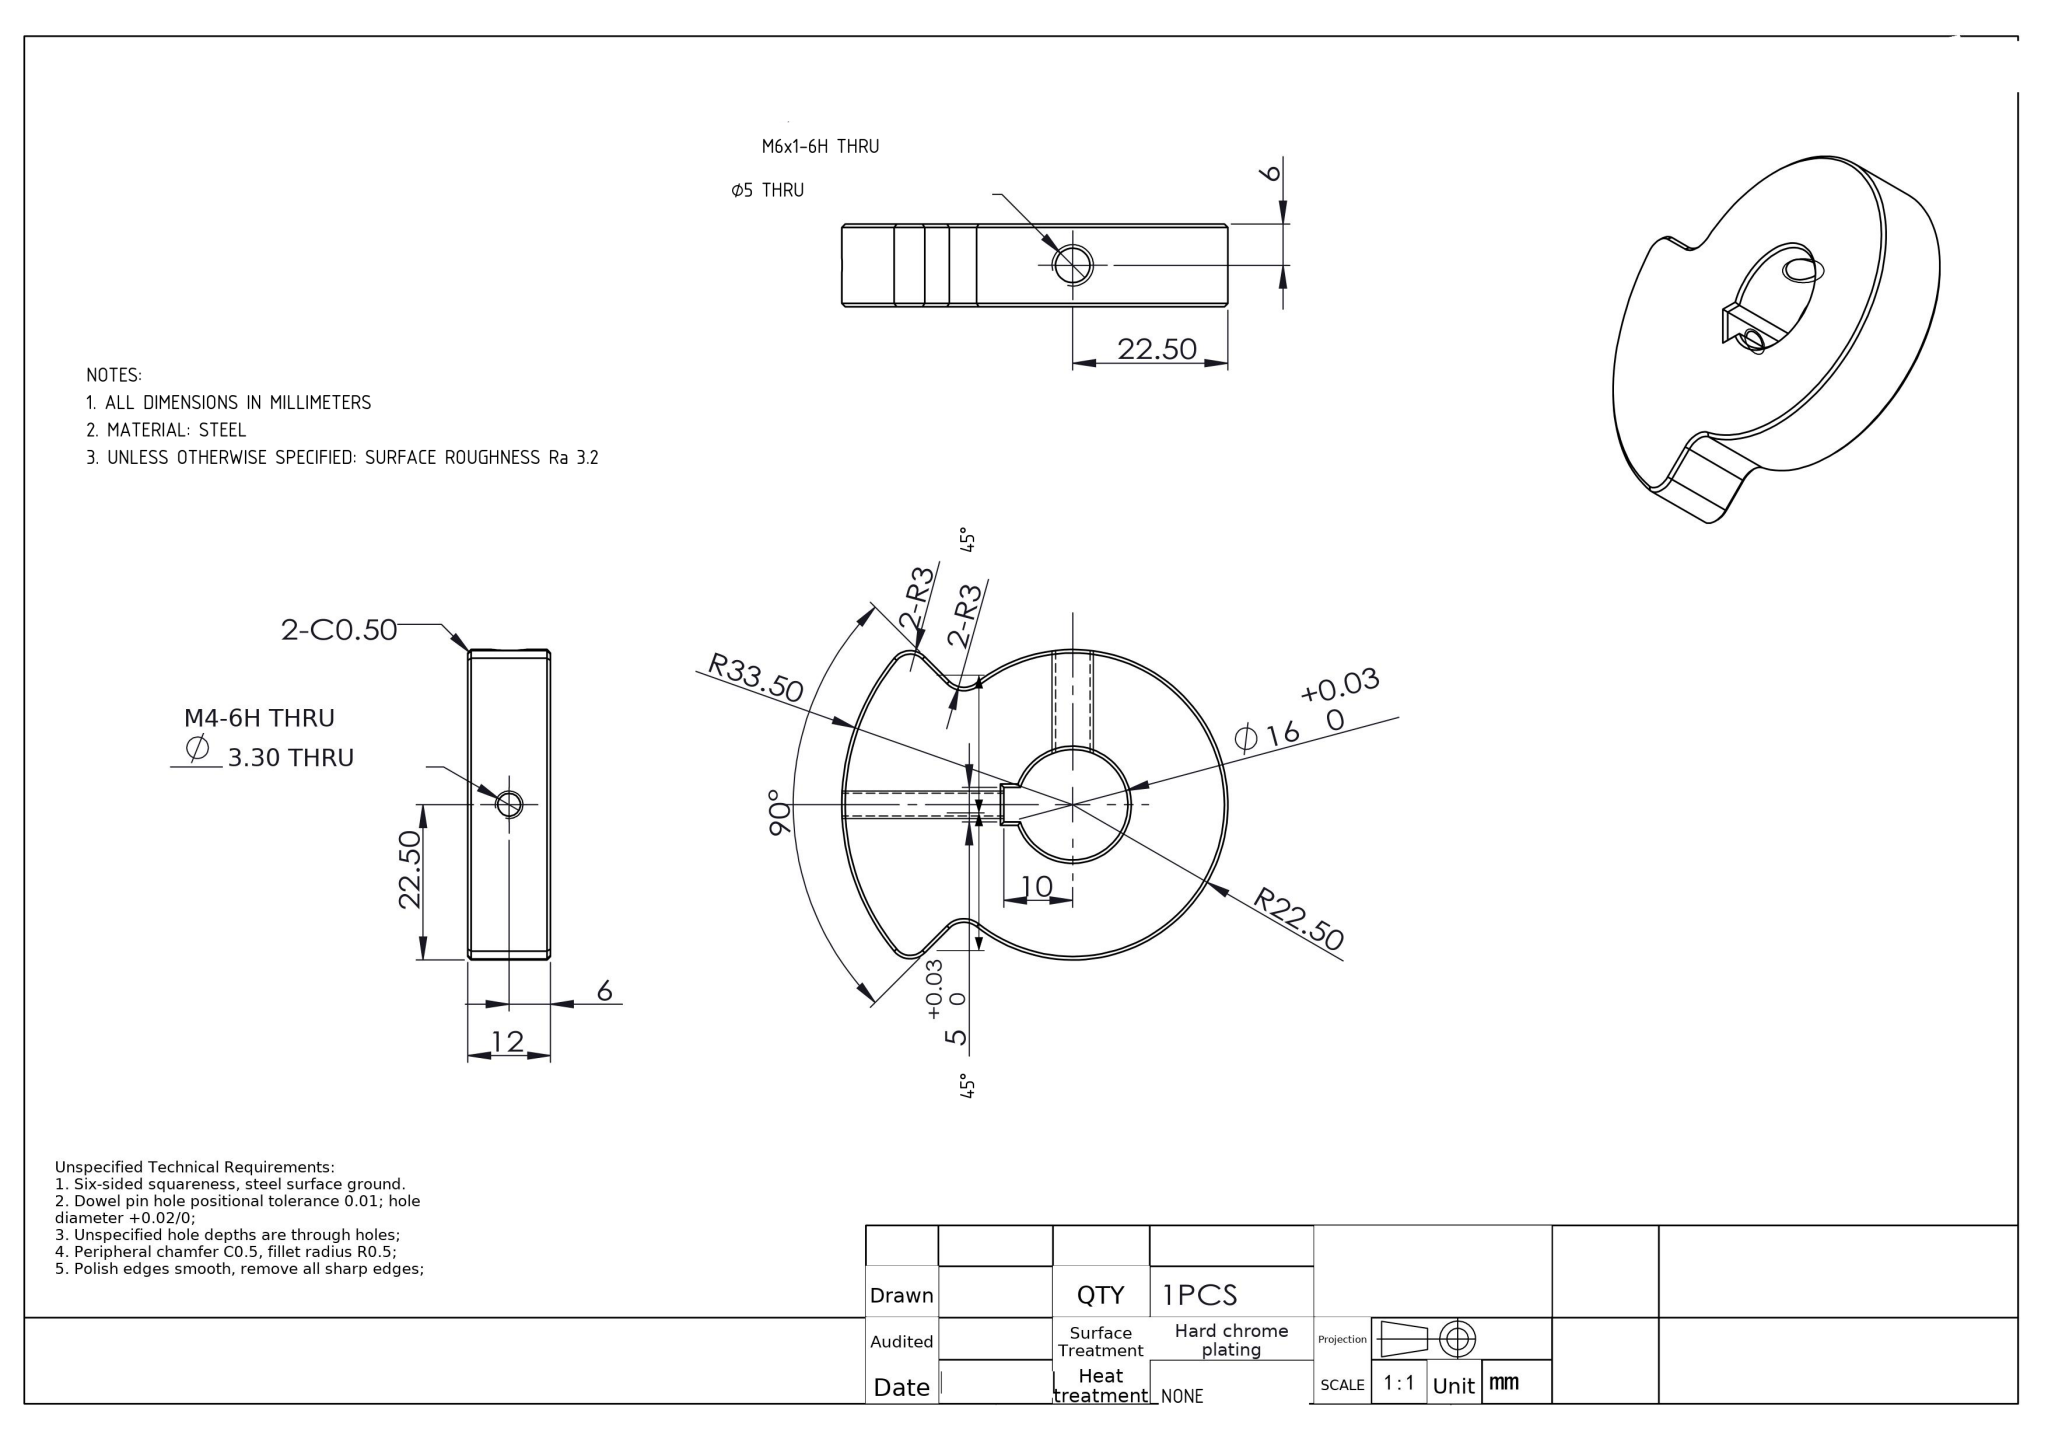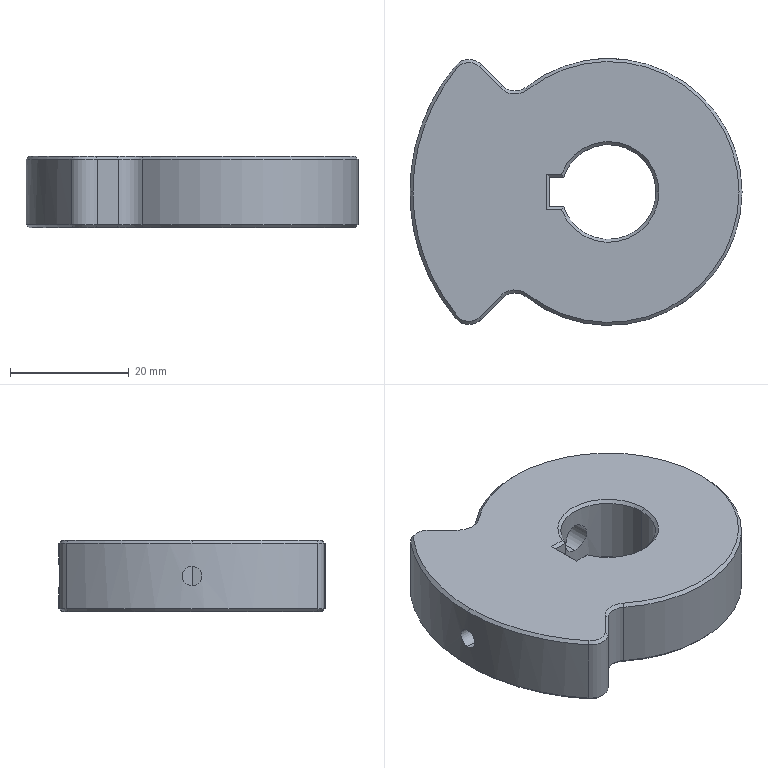Part | NX | mm | 1 solid | 47 faces | box 56 x 45 x 12 mm | volume 21790 mm3 | cone 17 | plane 17 | cylinder 13 | commonest cylinder face diameters 6 x4 3.3 x2 5 x2 45 x2 16 x2 67 x1